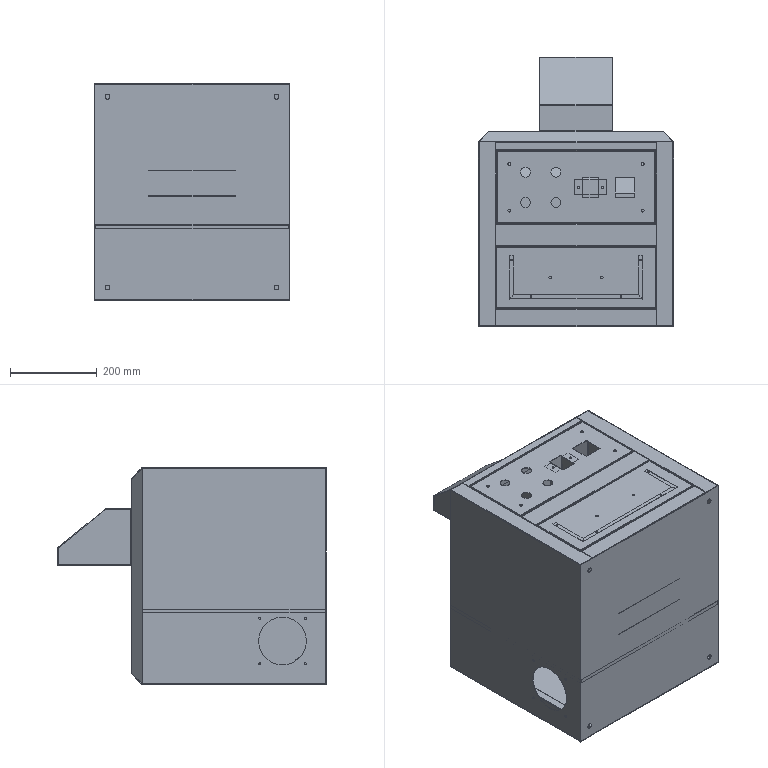Assembly | SolidWorks | mm | 42 component files | 42 solids | 1431 faces | box 451.7 x 620.2 x 500.38 mm | volume 2715264 mm3 | plane 1008 | cylinder 407 | spline 16 | commonest cylinder face diameters 0.2 x105 2.2 x58 2.6 x38 3 x32 6 x20 4.5 x20 7 x19 5 x18
Bill of materials:
CircuitBreakerBracket_2 | 1 |  | Thin formed sheet bracket with a hat-shaped profile: a deep U-channel with a flat base and two parallel side walls, each wall ending in an outward horizontal flange that has one round hole.
Drawer | 1 |  | Thin sheet shell with a U-shaped plan: a large rectangular back panel and two side panels. A narrow inward flange runs along the top edge. Each side panel has a vertical column of four small holes in two pairs, and the top flange has small holes.
DrawerPlate | 1 |  | Rectangular flat plate, thicker than the sheet parts. It has two larger round through-holes near the middle and four small holes in a staggered arrangement: two near the top corners and two lower and further inboard.
FrontPanel | 1 |  | Rectangular flat plate with many cutouts: four large round holes in a 2x2 grid, two rectangular openings of different sizes, a small hole on each side of the smaller rectangular opening, and four small holes near the corners.
Lampshade1 | 2 |  | Thin flat plate with a pentagon-like outline: one long straight edge, two edges that taper toward a shorter parallel end edge. A keyhole-shaped slot runs from the straight edge into a round hole near the middle, and there are two small holes near the straight edge.
Lampshade2 | 1 |  | Long formed sheet bracket. A raised central channel section runs between two offset end tabs, giving a hat-like side profile. Each end tab has two obround slots, and narrow lips run along the long edges of the central section.
Lampshade3 | 2 |  | Long, slender angle strip with an L-shaped section: two legs of unequal length joined by a rounded bend, and no visible holes.
Lampshade4 | 2 |  | Long, slender formed profile with a Z-like section: a horizontal top leg, a vertical web, and a lower leg angled away from the web. Both bends are rounded, and there are no visible holes.
Lampshade5 | 2 |  | Small L-shaped angle bracket with a rounded bend. The larger leg has two round through-holes in a line, and the shorter leg has no visible holes.
LampHolderMountingPlate | 2 |  | Tall L-shaped angle bracket with a rounded bend. One leg has a large central round hole with a small hole above and below it. The other leg has two small round holes.
LightBox1 | 1 |  | Thin sheet channel with a faceted section: a flat back face, two angled side faces, two flat side walls, and short return lips at the open side. The flat back face has two large round holes.
LightBox2 | 2 |  | Thin flat plate with a pentagon-like outline: a straight edge and tapered sides leading to a shorter end. A narrow flange appears to be bent along the straight edge, and there are two small round holes near the shorter end.
LightBoxBracket | 2 |  | L-shaped bent thin-plate angle bracket with a single round hole in the wider leg.
RearPanel | 1 |  | Shallow square tray: flat square plate with short raised walls on all four edges and four small holes near the corners.
AirDuct1 | 1 |  | Folded thin-wall enclosure shape with a sloped face: a flat base with a large circular cutout, side walls, and a partial top panel that steps down at an angle.
AirDuct2 | 1 |  | Flat thin plate shaped like a rectangle with one corner cut off diagonally (pentagon outline), with a narrow right-angle flange along one straight edge.
AirDuct3 | 1 |  | Flat thin plate shaped like a rectangle with one corner cut off diagonally (pentagon outline), with a narrow right-angle flange along one straight edge, on the opposite side from unnamed part.
BottomPlate | 1 |  | Square-ish flat panel with four corner holes, and short stepped (joggled) return flanges along two opposite edges.
CircuitBreakerBracket | 1 |  | Plain L-shaped angle: a roughly square main face with a narrow perpendicular flange along one edge, and no holes.
DrawerBox | 1 |  | U-shaped thin-wall channel (back wall plus two side walls), with four small holes in a line on one side wall.
DrawerBoxBracket | 1 |  | Long C-channel with a web, two equal parallel flanges and rounded bends; no holes.
FrontCrossbeam | 1 |  | Long hat-section (omega) profile: a raised central channel with two outward flat flanges and rounded bends.
LeftSidePanel | 1 |  | Large rectangular panel with stepped return flanges on the top and bottom edges, and one large circular opening near a lower corner, ringed by four small holes in a square pattern.
MountingAngle | 8 |  | Flat right-triangle plate (gusset-like shape) with one round through hole.
Partition | 1 |  | Thin flat, nearly square plate. Two corners on one edge are chamfered, that same edge has a rectangular notch near one end, and there is one elongated slot near the opposite edge.
RightSidePanel | 1 |  | Formed thin-walled panel: a near-square main web with short return flanges along two opposite edges. Each flange ends in a small inward-turned lip, giving a shallow C or hat-like profile in section. There is one round hole near one corner of the web.
Top | 1 |  | Formed tray-like panel: a near-square web with angled side walls on two opposite edges and stepped flanges along the other two edges. There is a rectangular cutout in the upper-central area and two small round holes, one near each side edge.
WireDuct | 1 |  | Straight, constant-section U-shaped channel with thin walls, a flat base and two parallel side legs. The inside corners are rounded. No holes or cutouts are visible.
Mates:
1. concentric | Lampshade-1/Lampshade2-1 face at (109.141, -16.087, 100) dir (0, 1, 0) r 2 | LightBox-1/LampHolderMountingPlate-2 face at (109.141, -15.087, 100) dir (0, 1, 0) r 1.25
2. concentric | WeldmentDrawing-1/Top-1 face at (158.141, 92.048, 80) dir (0, 1, 0) r 5 | LightBox-1/LightBoxBracket-2 face at (158.141, 28.413, 80) dir (0, 1, 0) r 5.5
3. concentric | WeldmentDrawing-1/Top-1 face at (-221.859, 92.048, 80) dir (0, 1, 0) r 5 | LightBox-1/LightBoxBracket-1 face at (-221.859, 28.413, 80) dir (0, 1, 0) r 5.5
4. parallel | Lampshade-1/Lampshade2-1 face at (-173.859, -16.087, 60) dir (0, 1, 0) r 2 | LightBox-1/LampHolderMountingPlate-1 face at (-172.859, -15.087, 60) dir (0, 1, 0) r 1.25
5. coincident | Lampshade-1/Lampshade2-1 face at (40.897, -15.087, 91.133) dir (0, 1, 0) | LightBox-1/LampHolderMountingPlate-2 face at (159.189, -15.087, 80.594) dir (0, -1, 0)
6. parallel | Lampshade-1/Lampshade1-1 face at (87.141, -36.087, 80) dir (1, 0, 0) | LightBox-1/LightBox2-1 face at (128.141, -24.733, 77.036) dir (1, 0, 0)
7. coincident | CircuitBreakerBracket_2-1 face at (19.433, -57.787, 249.183) dir (0, 0, 1) | FrontPanel-1 face at (-137.636, -20.961, 249.183) dir (0, 0, -1)
8. concentric | CircuitBreakerBracket_2-1 face at (29.64, -36.752, 248.183) dir (0, 0, 1) r 2.5 | FrontPanel-1 face at (29.64, -36.752, 249.183) dir (0, 0, 1) r 2.25
9. concentric | CircuitBreakerBracket_2-1 face at (-26.36, -36.752, 248.183) dir (0, 0, 1) r 2.5 | FrontPanel-1 face at (-26.36, -36.752, 249.183) dir (0, 0, 1) r 2.25
10. concentric | WeldmentDrawing-1/MountingAngle-2 face at (121.64, 16.748, 230) dir (0, 0, 1) r 4 | FrontPanel-1 face at (121.64, 16.748, 249.183) dir (0, 0, 1) r 3.5
11. concentric | WeldmentDrawing-1/MountingAngle-3 face at (-185.36, 16.748, 230) dir (0, 0, 1) r 4 | FrontPanel-1 face at (-185.36, 16.748, 249.183) dir (0, 0, 1) r 3.5
12. distance | DrawerWelding-1/DrawerPlate-1 face at (151.64, -226.356, 249.95) dir (1, 0, 0) | WeldmentDrawing-1/RightSidePanel-1 face at (153.14, -316.781, 195.572) dir (-1, 0, 0)
13. distance | DrawerWelding-1/DrawerPlate-1 face at (-122.832, -315.452, 249.95) dir (0, -1, 0) | WeldmentDrawing-1/BottomPlate-1 face at (-195.03, -316.952, 185.339) dir (0, 1, 0)
14. concentric | WeldmentDrawing-1/MountingAngle-8 face at (121.64, 16.748, -231.2) dir (0, 0, 1) r 4 | RearPanel-1 face at (121.64, 16.748, -248.474) dir (0, 0, -1) r 3.5
15. concentric | WeldmentDrawing-1/MountingAngle-5 face at (-185.36, 16.748, -231.2) dir (0, 0, 1) r 4 | RearPanel-1 face at (-185.36, 16.748, -248.474) dir (0, 0, -1) r 3.5
16. coincident | Drawer-1 face at (-169.764, -65.114, 160) dir (0, 0, 1) | DrawerPlate-1 face at (-173.944, 1.982, 160) dir (0, 0, -1)
17. concentric | Drawer-1 face at (-231.473, 23.886, 159) dir (0, 0, 1) r 1.5 | DrawerPlate-1 face at (-231.473, 23.886, 160) dir (0, 0, 1) r 1.5
18. concentric | Drawer-1 face at (21.527, -60.114, 159) dir (0, 0, 1) r 1.5 | DrawerPlate-1 face at (21.527, -60.114, 160) dir (0, 0, 1) r 1.5
19. coincident | Lampshade2-1 face at (-21.408, 18.767, 46.244) dir (0, 0, -1) | Lampshade1-1 face at (-10.275, -27.233, 46.244) dir (0, 0, 1)
20. coincident | Lampshade2-1 face at (-21.408, 18.767, -196.756) dir (0, 0, 1) | Lampshade1-2 face at (-10.275, -27.233, -196.756) dir (0, 0, -1)
21. coincident | Lampshade2-1 face at (-21.408, 17.767, 0) dir (0, -1, 0) | Lampshade1-1 face at (9.725, 17.767, 44.744) dir (0, 1, 0)
22. coincident | Lampshade2-1 face at (-21.408, 17.767, 0) dir (0, -1, 0) | Lampshade1-2 face at (9.725, 17.767, -196.756) dir (0, 1, 0)
23. distance | Lampshade1-1 face at (61.225, -82.233, 44.744) dir (1, 0, 0) | Lampshade2-1 face at (28.725, 18.767, 0) dir (1, 0, 0)
24. coincident | Lampshade1-1 face at (61.225, -82.233, 44.744) dir (1, 0, 0) | Lampshade1-2 face at (61.225, -82.233, -196.756) dir (1, 0, 0)
25. coincident | Lampshade1-1 face at (61.225, -82.233, 44.744) dir (1, 0, 0) | Lampshade3-2 face at (61.225, -67.233, -195.256) dir (1, 0, 0)
26. coincident | Lampshade1-1 face at (-0.2752, -82.233, 44.744) dir (0, -1, 0) | Lampshade3-2 face at (61.225, -82.233, -195.256) dir (0, -1, 0)
27. coincident | Lampshade1-1 face at (-10.275, -27.233, 44.744) dir (0, 0, -1) | Lampshade3-2 face at (60.225, -81.133, 44.744) dir (0, 0, 1)
28. coincident | Lampshade1-1 face at (-81.775, -62.233, 44.744) dir (-1, 0, 0) | Lampshade3-1 face at (-81.775, -67.233, 44.744) dir (-1, 0, 0)
29. coincident | Lampshade1-1 face at (-81.775, -82.233, 44.744) dir (0, -1, 0) | Lampshade3-1 face at (-81.775, -82.233, 44.744) dir (0, -1, 0)
30. coincident | Lampshade1-1 face at (-10.275, -27.233, 44.744) dir (0, 0, -1) | Lampshade3-1 face at (-80.675, -81.133, 44.744) dir (0, 0, 1)
31. distance | Lampshade4-2 face at (14.725, -1.233, -195.256) dir (1, 0, 0) | Lampshade3-2 face at (61.225, -67.233, -195.256) dir (1, 0, 0)
32. distance | Lampshade4-1 face at (-35.275, -1.233, 44.744) dir (-1, 0, 0) | Lampshade3-1 face at (-81.775, -67.233, 44.744) dir (-1, 0, 0)
33. distance | Lampshade4-1 face at (-35.275, -11.233, 44.744) dir (0, -1, 0) | Lampshade3-1 face at (-81.775, -82.233, 44.744) dir (0, -1, 0)
34. coincident | Lampshade4-1 face at (-35.275, -11.233, 44.744) dir (0, -1, 0) | Lampshade4-2 face at (14.725, -11.233, -195.256) dir (0, -1, 0)
35. coincident | Lampshade4-1 face at (-24.496, -11.883, 44.744) dir (0, 0, 1) | Lampshade4-2 face at (13.725, -10.133, 44.744) dir (0, 0, 1)
36. coincident | Lampshade1-1 face at (-10.275, -27.233, 44.744) dir (0, 0, -1) | Lampshade4-1 face at (-24.496, -11.883, 44.744) dir (0, 0, 1)
37. coincident | Lampshade1-1 face at (-10.275, -27.233, 46.244) dir (0, 0, 1) | Lampshade5-1 face at (66.122, -65.733, 46.244) dir (0, 0, -1)
38. distance | Lampshade5-1 face at (43.225, -67.233, 76.244) dir (1, 0, 0) | Lampshade3-2 face at (61.225, -67.233, -195.256) dir (1, 0, 0)
39. distance | Lampshade5-1 face at (66.122, -67.233, 21.162) dir (0, -1, 0) | Lampshade3-2 face at (61.225, -82.233, -195.256) dir (0, -1, 0)
40. coincident | Lampshade1-2 face at (-10.275, -27.233, -196.756) dir (0, 0, -1) | Lampshade5-2 face at (-4.672, -65.733, -196.756) dir (0, 0, 1)
41. coincident | Lampshade5-1 face at (66.122, -67.233, 21.162) dir (0, -1, 0) | Lampshade5-2 face at (-4.672, -67.233, -171.674) dir (0, -1, 0)
42. coincident | Lampshade5-1 face at (43.225, -67.233, 76.244) dir (1, 0, 0) | Lampshade5-2 face at (43.225, -57.233, -196.756) dir (1, 0, 0)
43. coincident | LightBox1-1 face at (-148.852, 56.327, 59.32) dir (-1, 0, 0) | LightBox2-2 face at (-148.852, 2.681, 12.964) dir (1, 0, 0)
44. coincident | LightBox1-1 face at (169.148, -72.673, 100) dir (0, 0, 1) | LightBox2-2 face at (-148.852, -22.673, 100) dir (0, 0, 1)
45. coincident | LightBox1-1 face at (-148.852, -72.673, 34.468) dir (0, -1, 0) | LightBox2-2 face at (-149.852, -72.673, 12.964) dir (0, -1, 0)
46. coincident | LightBox1-1 face at (169.148, -22.932, 99) dir (1, 0, 0) | LightBox2-1 face at (169.148, 2.681, 7.036) dir (-1, 0, 0)
47. coincident | LightBox1-1 face at (169.148, -72.673, 100) dir (0, 0, 1) | LightBox2-1 face at (169.148, -72.673, 100) dir (0, 0, 1)
48. coincident | LightBox1-1 face at (-148.852, -72.673, 34.468) dir (0, -1, 0) | LightBox2-1 face at (170.148, -72.673, 7.036) dir (0, -1, 0)
49. concentric | LightBox2-1 face at (169.148, 22.327, 30) dir (1, 0, 0) r 1.5 | LampHolderMountingPlate-2 face at (167.648, 22.327, 30) dir (1, 0, 0) r 1.5
50. concentric | LightBox2-1 face at (169.148, 22.327, -10) dir (1, 0, 0) r 1.5 | LampHolderMountingPlate-2 face at (167.648, 22.327, -10) dir (1, 0, 0) r 1.5
51. coincident | LightBox2-1 face at (169.148, 2.681, 7.036) dir (-1, 0, 0) | LampHolderMountingPlate-2 face at (169.148, 13.827, 10.594) dir (1, 0, 0)
52. concentric | LightBox2-2 face at (-148.852, 22.327, 30) dir (-1, 0, 0) r 1.5 | LampHolderMountingPlate-1 face at (-147.352, 22.327, 30) dir (-1, 0, 0) r 1.5
53. concentric | LightBox2-2 face at (-148.852, 22.327, -10) dir (-1, 0, 0) r 1.5 | LampHolderMountingPlate-1 face at (-147.352, 22.327, -10) dir (-1, 0, 0) r 1.5
54. coincident | LightBox2-2 face at (-148.852, 2.681, 12.964) dir (1, 0, 0) | LampHolderMountingPlate-1 face at (-148.852, 13.827, 9.406) dir (-1, 0, 0)
55. coincident | LightBox1-1 face at (169.148, 57.327, 60) dir (0, 1, 0) | LightBoxBracket-1 face at (-203.628, 57.327, 21.9) dir (0, 1, 0)
56. coincident | LightBox2-2 face at (-149.852, 2.681, 12.964) dir (-1, 0, 0) | LightBoxBracket-1 face at (-149.852, 57.327, 21.9) dir (1, 0, 0)
57. distance | LightBoxBracket-1 face at (-149.852, 55.827, 60) dir (0, 0, 1) | LightBox1-1 face at (169.148, -72.673, 100) dir (0, 0, 1)
58. coincident | LightBoxBracket-1 face at (-203.628, 57.327, 21.9) dir (0, 1, 0) | LightBoxBracket-2 face at (223.923, 57.327, -1.9) dir (0, 1, 0)
59. coincident | LightBox2-1 face at (170.148, 2.681, 7.036) dir (1, 0, 0) | LightBoxBracket-2 face at (170.148, 57.327, -1.9) dir (-1, 0, 0)
60. coincident | LightBoxBracket-1 face at (-194.852, 55.827, -40) dir (0, 0, -1) | LightBoxBracket-2 face at (215.148, 55.827, -40) dir (0, 0, -1)
61. coincident | BottomPlate-1 face at (-230.38, -176.974, 250) dir (0, 0, 1) | RightSidePanel-1 face at (157.789, -138.003, 250) dir (0, 0, 1)
62. coincident | BottomPlate-1 face at (-230.38, -176.974, 185.339) dir (0, 1, 0) | RightSidePanel-1 face at (156.589, -176.974, 250) dir (0, -1, 0)
63. coincident | BottomPlate-1 face at (157.789, -178.174, 250) dir (1, 0, 0) | RightSidePanel-1 face at (157.789, -138.003, 195.571) dir (1, 0, 0)
64. coincident | BottomPlate-1 face at (-230.38, -176.974, 250) dir (0, 0, 1) | LeftSidePanel-1 face at (-291.011, -143.384, 250) dir (0, 0, 1)
65. coincident | BottomPlate-1 face at (-230.38, -176.974, 185.339) dir (0, 1, 0) | LeftSidePanel-1 face at (-252.211, -176.974, 250) dir (0, -1, 0)
66. coincident | BottomPlate-1 face at (-292.211, -178.174, 250) dir (-1, 0, 0) | LeftSidePanel-1 face at (-292.211, -143.384, 169.821) dir (-1, 0, 0)
67. coincident | Top-1 face at (-199.522, 272.377, 250) dir (0, 0, 1) | RightSidePanel-1 face at (157.789, -138.003, 250) dir (0, 0, 1)
68. coincident | Top-1 face at (117.789, 227.026, 250) dir (1, 0, 0) | RightSidePanel-1 face at (117.789, -138.003, 195.571) dir (-1, 0, 0)
69. distance | Top-1 face at (-252.208, 208.226, 230) dir (0, -1, 0) | LeftSidePanel-1 face at (-233.411, 207.826, 230) dir (0, 1, 0)
70. coincident | LeftSidePanel-1 face at (-291.011, -143.384, 250) dir (0, 0, 1) | FrontCrossbeam-1 face at (-176.882, 9.582, 250) dir (0, 0, 1)
71. coincident | RightSidePanel-1 face at (117.789, -138.003, 195.571) dir (-1, 0, 0) | FrontCrossbeam-1 face at (117.789, 56.826, 248.8) dir (1, 0, 0)
72. distance | RightSidePanel-1 face at (86.007, 75.826, 231.4) dir (0, -1, 0) | FrontCrossbeam-1 face at (117.789, 75.626, 230) dir (0, 1, 0)
73. coincident | BottomPlate-1 face at (-230.38, -176.974, 185.339) dir (0, 1, 0) | DrawerBoxBracket-1 face at (-167.211, -176.974, -10) dir (0, -1, 0)
74. distance | DrawerBoxBracket-1 face at (32.789, -121.574, 50) dir (1, 0, 0) | RightSidePanel-1 face at (157.789, -138.003, 195.571) dir (1, 0, 0)
75. distance | DrawerBoxBracket-1 face at (-96.889, -120.374, 50) dir (0, 0, 1) | BottomPlate-1 face at (-230.38, -176.974, 250) dir (0, 0, 1)
76. coincident | BottomPlate-1 face at (117.789, -119.374, 230) dir (0, 1, 0) | DrawerBox-1 face at (-178.758, -119.374, 177.531) dir (0, 1, 0)
77. distance | DrawerBox-1 face at (-233.711, -119.374, 177.531) dir (1, 0, 0) | LeftSidePanel-1 face at (-233.411, -118.974, 230) dir (1, 0, 0)
78. coincident | RightSidePanel-1 face at (157.789, -138.003, 230) dir (0, 0, -1) | DrawerBox-1 face at (-234.711, -120.374, 230) dir (0, 0, 1)
79. coincident | Partition-1 face at (-200.711, 240.026, -76) dir (-1, 0, 0) | WireDuct-1 face at (-200.711, 241.026, -35.082) dir (1, 0, 0)
80. coincident | Partition-1 face at (-245.711, 240.026, -76) dir (0, 1, 0) | WireDuct-1 face at (-207.176, 240.026, -35.082) dir (0, -1, 0)
81. distance | Partition-1 face at (-290.711, 246.75, -75) dir (-1, 0, 0) | LeftSidePanel-1 face at (-292.211, -143.384, 169.821) dir (-1, 0, 0)
82. coincident | DrawerBox-1 face at (-234.711, -120.374, -75) dir (0, 0, -1) | Partition-1 face at (-233.888, 246.75, -75) dir (0, 0, 1)
83. coincident | BottomPlate-1 face at (-230.38, -176.974, 185.339) dir (0, 1, 0) | Partition-1 face at (-233.888, -176.974, -75) dir (0, -1, 0)
84. distance | WireDuct-1 face at (-245.711, 240.026, -200) dir (0, 0, -1) | LeftSidePanel-1 face at (-291.011, -143.384, -250) dir (0, 0, -1)
85. coincident | Partition-1 face at (-233.888, 246.75, -76) dir (0, 0, -1) | CircuitBreakerBracket-1 face at (57.932, -18.474, -76) dir (0, 0, 1)
86. distance | CircuitBreakerBracket-1 face at (107.789, -19.974, -176) dir (1, 0, 0) | RightSidePanel-1 face at (157.789, -138.003, 195.571) dir (1, 0, 0)
87. distance | CircuitBreakerBracket-1 face at (57.932, -18.474, -128.034) dir (0, 1, 0) | Partition-1 face at (39.789, -68.474, -76) dir (0, -1, 0)
88. coincident | LeftSidePanel-1 face at (-233.411, -118.974, 230) dir (1, 0, 0) | MountingAngle-4 face at (-233.411, 115.626, 230) dir (-1, 0, 0)
89. coincident | FrontCrossbeam-1 face at (117.789, 75.626, 230) dir (0, 1, 0) | MountingAngle-4 face at (-233.411, 75.626, 230) dir (0, -1, 0)
90. coincident | LeftSidePanel-1 face at (-291.011, -143.384, 231.2) dir (0, 0, 1) | MountingAngle-4 face at (-193.569, 59.297, 231.2) dir (0, 0, 1)
91. coincident | LeftSidePanel-1 face at (-291.011, -143.384, 231.2) dir (0, 0, 1) | MountingAngle-3 face at (-249.74, 168.384, 231.2) dir (0, 0, 1)
92. coincident | LeftSidePanel-1 face at (-233.411, -118.974, 230) dir (1, 0, 0) | MountingAngle-3 face at (-233.411, 208.226, 230) dir (-1, 0, 0)
93. coincident | Top-1 face at (-252.208, 208.226, 230) dir (0, -1, 0) | MountingAngle-3 face at (-193.411, 208.226, 230) dir (0, 1, 0)
94. coincident | RightSidePanel-1 face at (98.989, 207.826, 230) dir (-1, 0, 0) | MountingAngle-1 face at (98.989, 75.626, 230) dir (1, 0, 0)
95. coincident | FrontCrossbeam-1 face at (117.789, 75.626, 230) dir (0, 1, 0) | MountingAngle-1 face at (58.989, 75.626, 230) dir (0, -1, 0)
96. coincident | RightSidePanel-1 face at (157.789, -138.003, 231.2) dir (0, 0, 1) | MountingAngle-1 face at (115.318, 115.467, 231.2) dir (0, 0, 1)
97. coincident | RightSidePanel-1 face at (98.989, 207.826, 230) dir (-1, 0, 0) | MountingAngle-2 face at (98.989, 168.226, 230) dir (1, 0, 0)
98. coincident | Top-1 face at (-252.208, 208.226, 230) dir (0, -1, 0) | MountingAngle-2 face at (98.989, 208.226, 230) dir (0, 1, 0)
99. coincident | Top-1 face at (-199.522, 272.026, 231.2) dir (0, 0, 1) | MountingAngle-2 face at (59.147, 224.554, 231.2) dir (0, 0, 1)
100. coincident | LeftSidePanel-1 face at (-291.011, -143.384, -231.2) dir (0, 0, -1) | MountingAngle-7 face at (-193.569, -135.703, -231.2) dir (0, 0, -1)
101. coincident | LeftSidePanel-1 face at (-233.411, 207.826, -230) dir (1, 0, 0) | MountingAngle-7 face at (-233.411, -79.374, -231.2) dir (-1, 0, 0)
102. coincident | BottomPlate-1 face at (-252.211, -119.374, -230) dir (0, 1, 0) | MountingAngle-7 face at (-233.411, -119.374, -231.2) dir (0, -1, 0)
103. coincident | Top-1 face at (-199.522, 272.026, -231.2) dir (0, 0, -1) | MountingAngle-5 face at (-249.74, 168.384, -231.2) dir (0, 0, -1)
104. coincident | Top-1 face at (117.789, 208.226, -230) dir (0, -1, 0) | MountingAngle-5 face at (-193.411, 208.226, -231.2) dir (0, 1, 0)
105. coincident | LeftSidePanel-1 face at (-233.411, 207.826, -230) dir (1, 0, 0) | MountingAngle-5 face at (-233.411, 208.226, -231.2) dir (-1, 0, 0)
106. coincident | RightSidePanel-1 face at (157.789, -138.003, -231.2) dir (0, 0, -1) | MountingAngle-8 face at (59.147, 224.554, -231.2) dir (0, 0, -1)
107. coincident | RightSidePanel-1 face at (98.989, -118.974, -230) dir (-1, 0, 0) | MountingAngle-8 face at (98.989, 168.226, -231.2) dir (1, 0, 0)
108. coincident | Top-1 face at (117.789, 208.226, -230) dir (0, -1, 0) | MountingAngle-8 face at (98.989, 208.226, -231.2) dir (0, 1, 0)
109. coincident | RightSidePanel-1 face at (157.789, -138.003, -231.2) dir (0, 0, -1) | MountingAngle-6 face at (115.318, -79.533, -231.2) dir (0, 0, -1)
110. coincident | RightSidePanel-1 face at (98.989, -118.974, -230) dir (-1, 0, 0) | MountingAngle-6 face at (98.989, -119.374, -231.2) dir (1, 0, 0)
111. coincident | BottomPlate-1 face at (-252.211, -119.374, -230) dir (0, 1, 0) | MountingAngle-6 face at (58.989, -119.374, -231.2) dir (0, -1, 0)
112. coincident | AirDuct1-1 face at (-151.21, 332.026, 155) dir (0, 0, 1) | AirDuct2-1 face at (-151.21, 272.026, 155) dir (0, 0, 1)
113. coincident | AirDuct1-1 face at (16.79, 272.026, 43.882) dir (0, -1, 0) | AirDuct2-1 face at (-152.21, 272.026, 63.971) dir (0, -1, 0)
114. coincident | AirDuct1-1 face at (-151.21, 331.697, 153.977) dir (-1, 0, 0) | AirDuct2-1 face at (-151.21, 344.871, 63.971) dir (1, 0, 0)
115. coincident | AirDuct1-1 face at (16.79, 272.026, 43.882) dir (0, -1, 0) | AirDuct3-1 face at (17.79, 272.026, 63.971) dir (0, -1, 0)
116. coincident | AirDuct1-1 face at (16.79, 331.633, 153.9) dir (1, 0, 0) | AirDuct3-1 face at (16.79, 344.871, 63.971) dir (-1, 0, 0)
117. coincident | AirDuct1-1 face at (-151.21, 332.026, 155) dir (0, 0, 1) | AirDuct3-1 face at (16.79, 272.026, 155) dir (0, 0, 1)
118. coincident | Top-1 face at (-199.522, 272.026, 144.932) dir (0, 1, 0) | AirDuct1-1 face at (16.79, 272.026, 43.882) dir (0, -1, 0)
119. coincident | Top-1 face at (-132.21, 270.826, 135) dir (0, 0, -1) | AirDuct1-1 face at (16.79, 272.026, 135) dir (0, 0, -1)
120. coincident | Top-1 face at (-2.21, 270.826, 135) dir (-1, 0, 0) | AirDuct3-1 face at (-2.21, 272.026, 45) dir (-1, 0, 0)